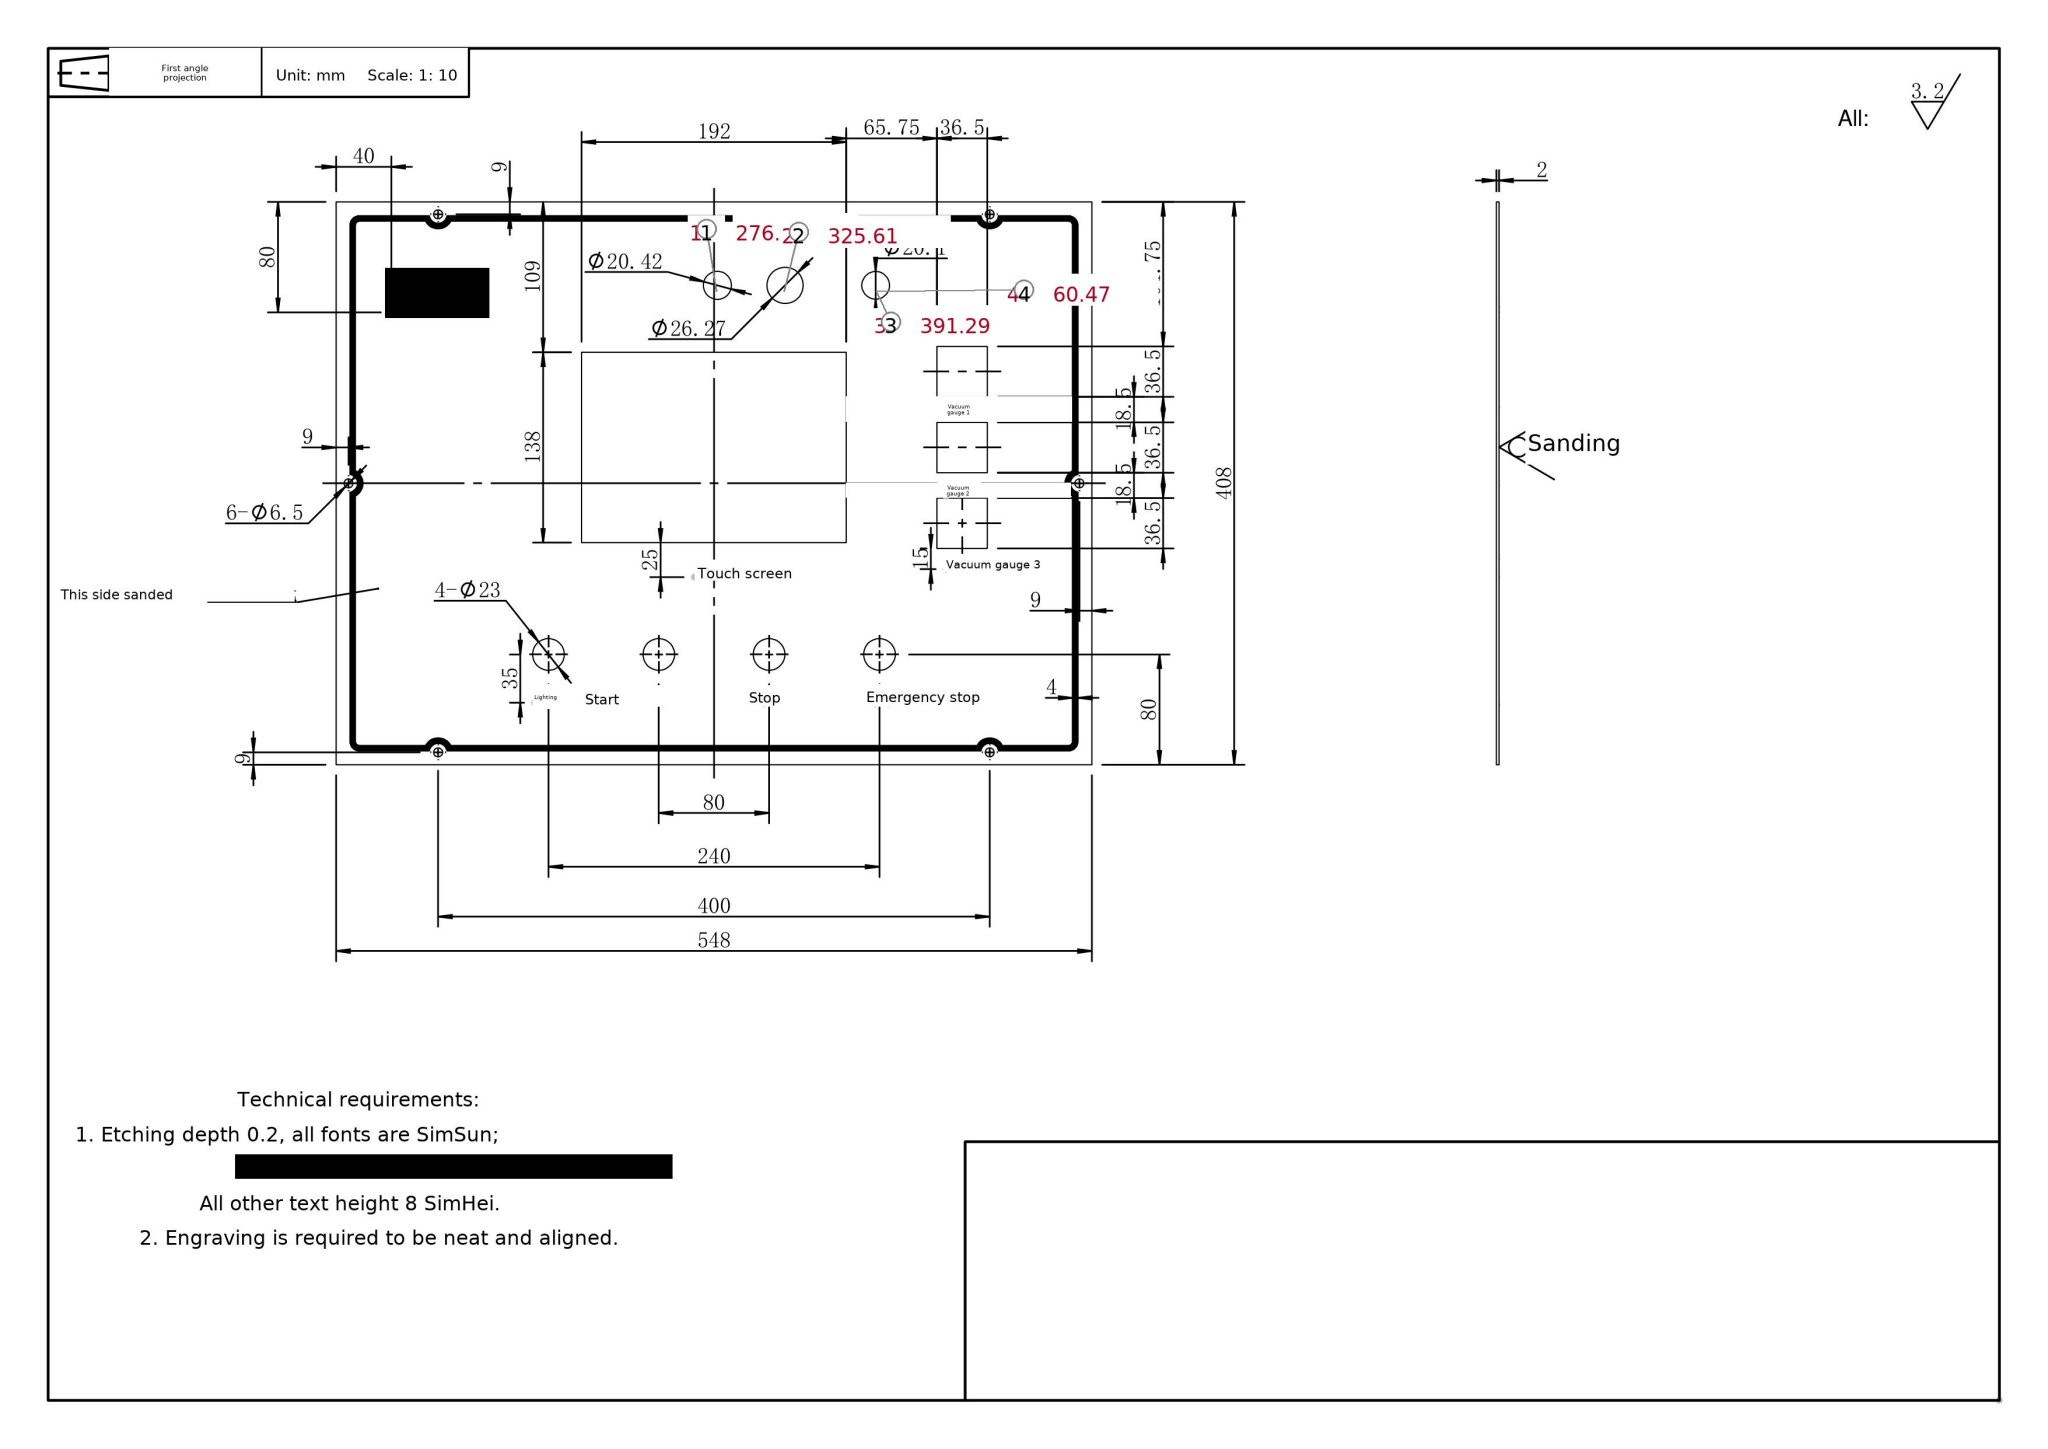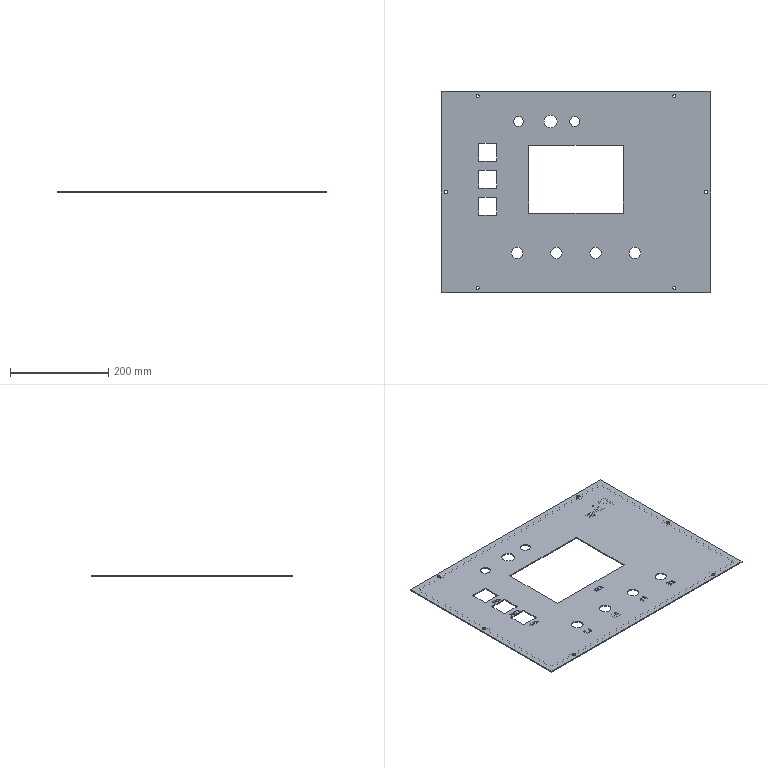Part | SolidWorks | mm | 1 solid | 2279 faces | box 548 x 408 x 2 mm | volume 378207 mm3 | plane 1642 | spline 589 | cylinder 48 | commonest cylinder face diameters 6.5 x12 23 x8 21 x7 13 x7 14 x4 6 x4 20.415 x2 20.096 x2